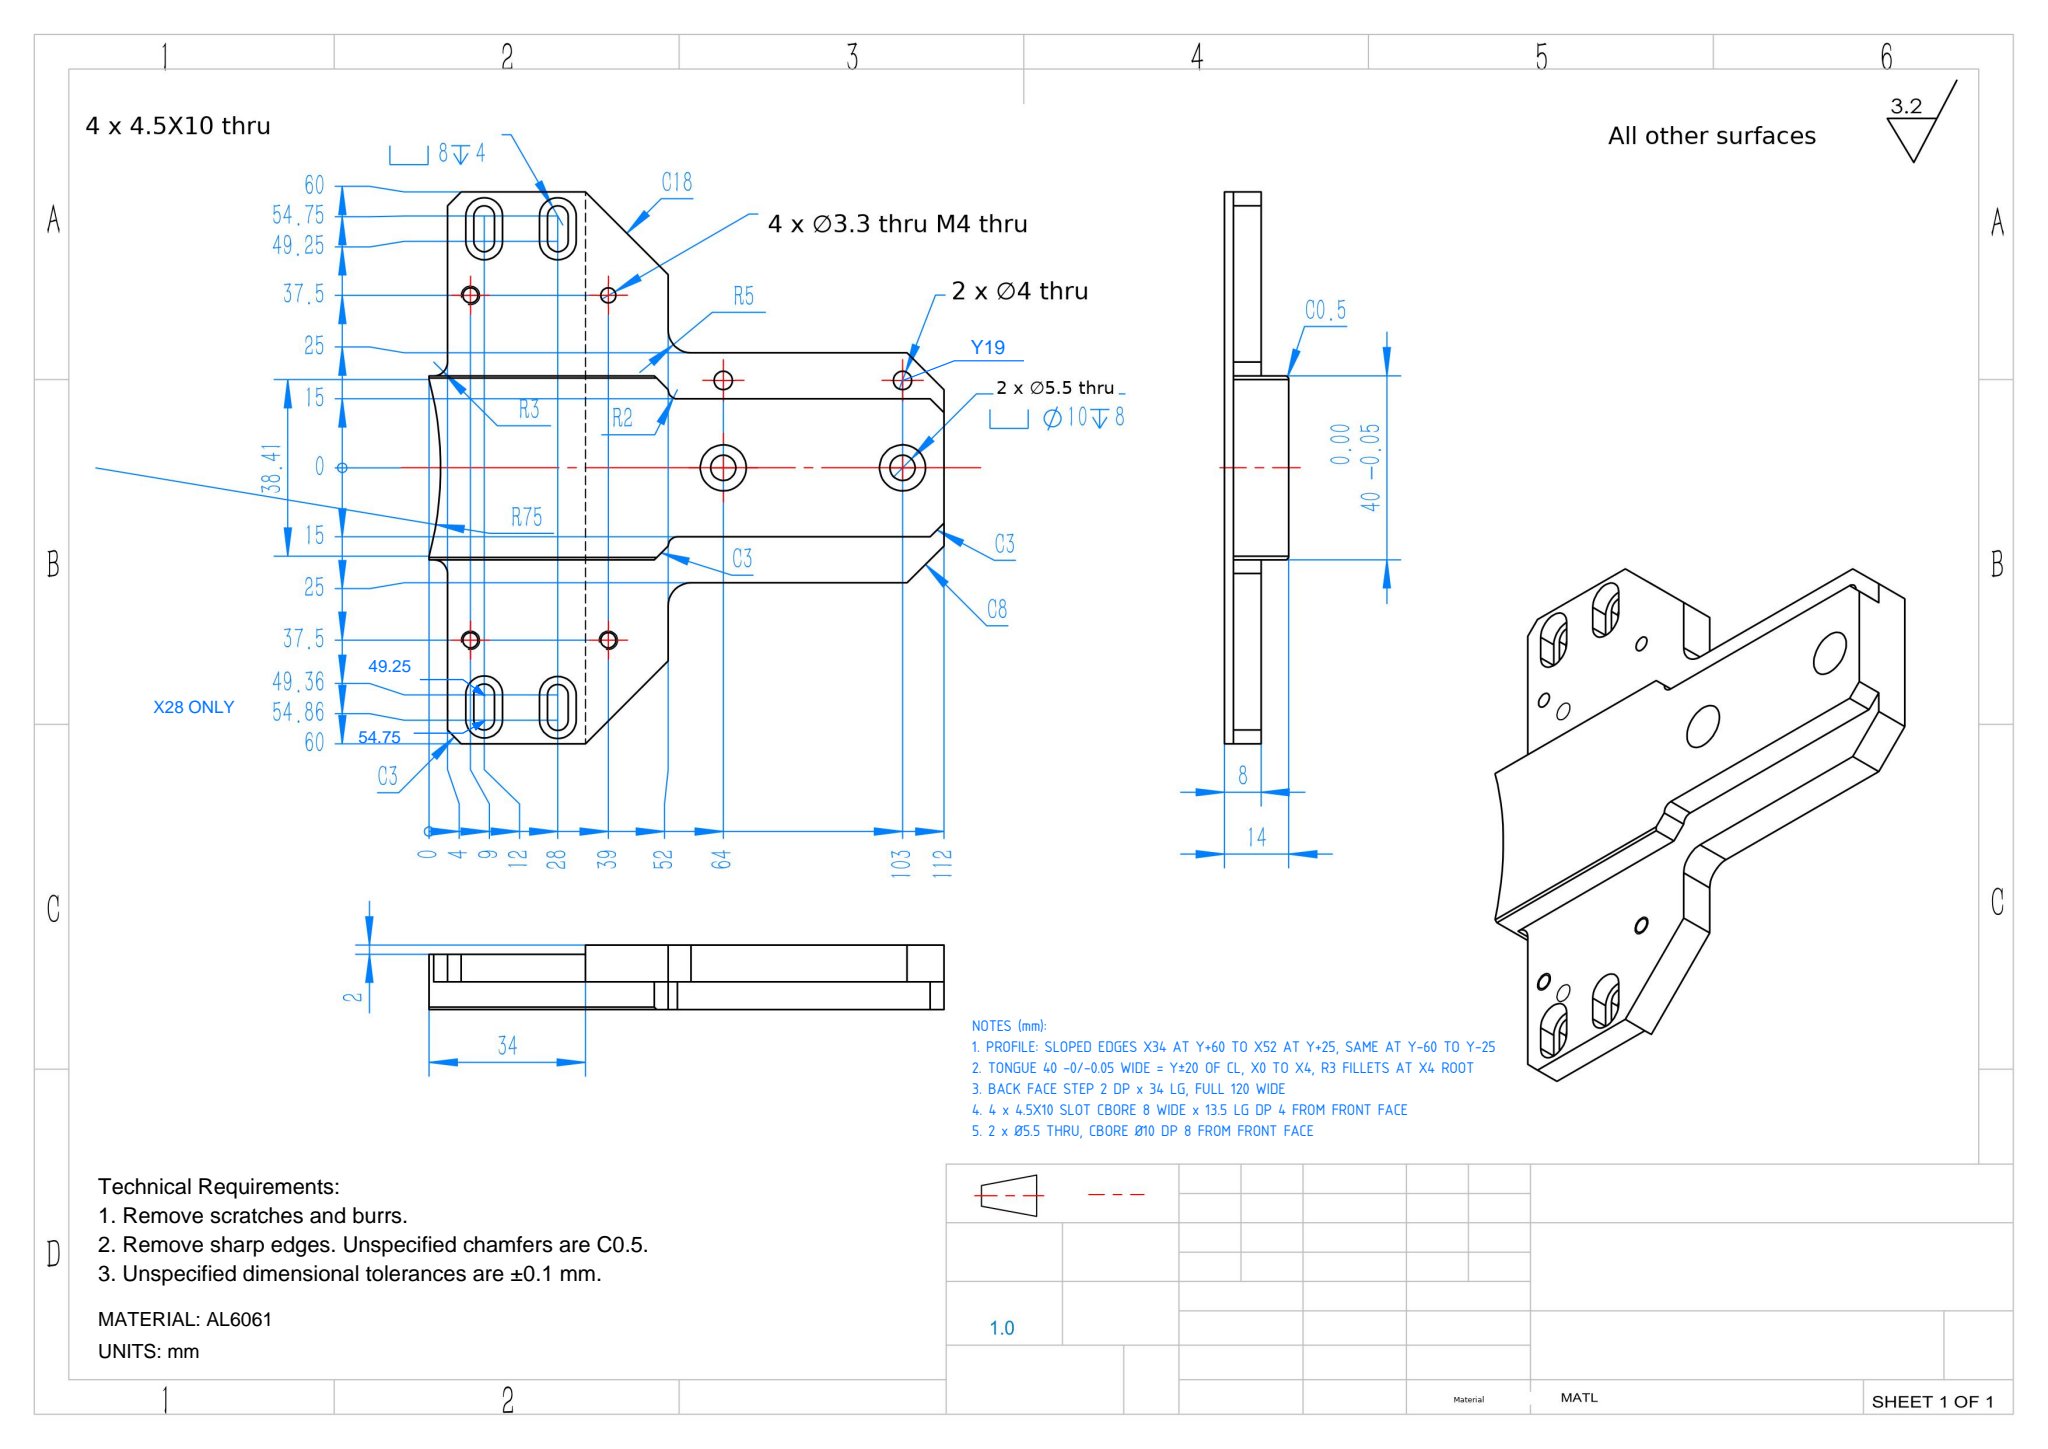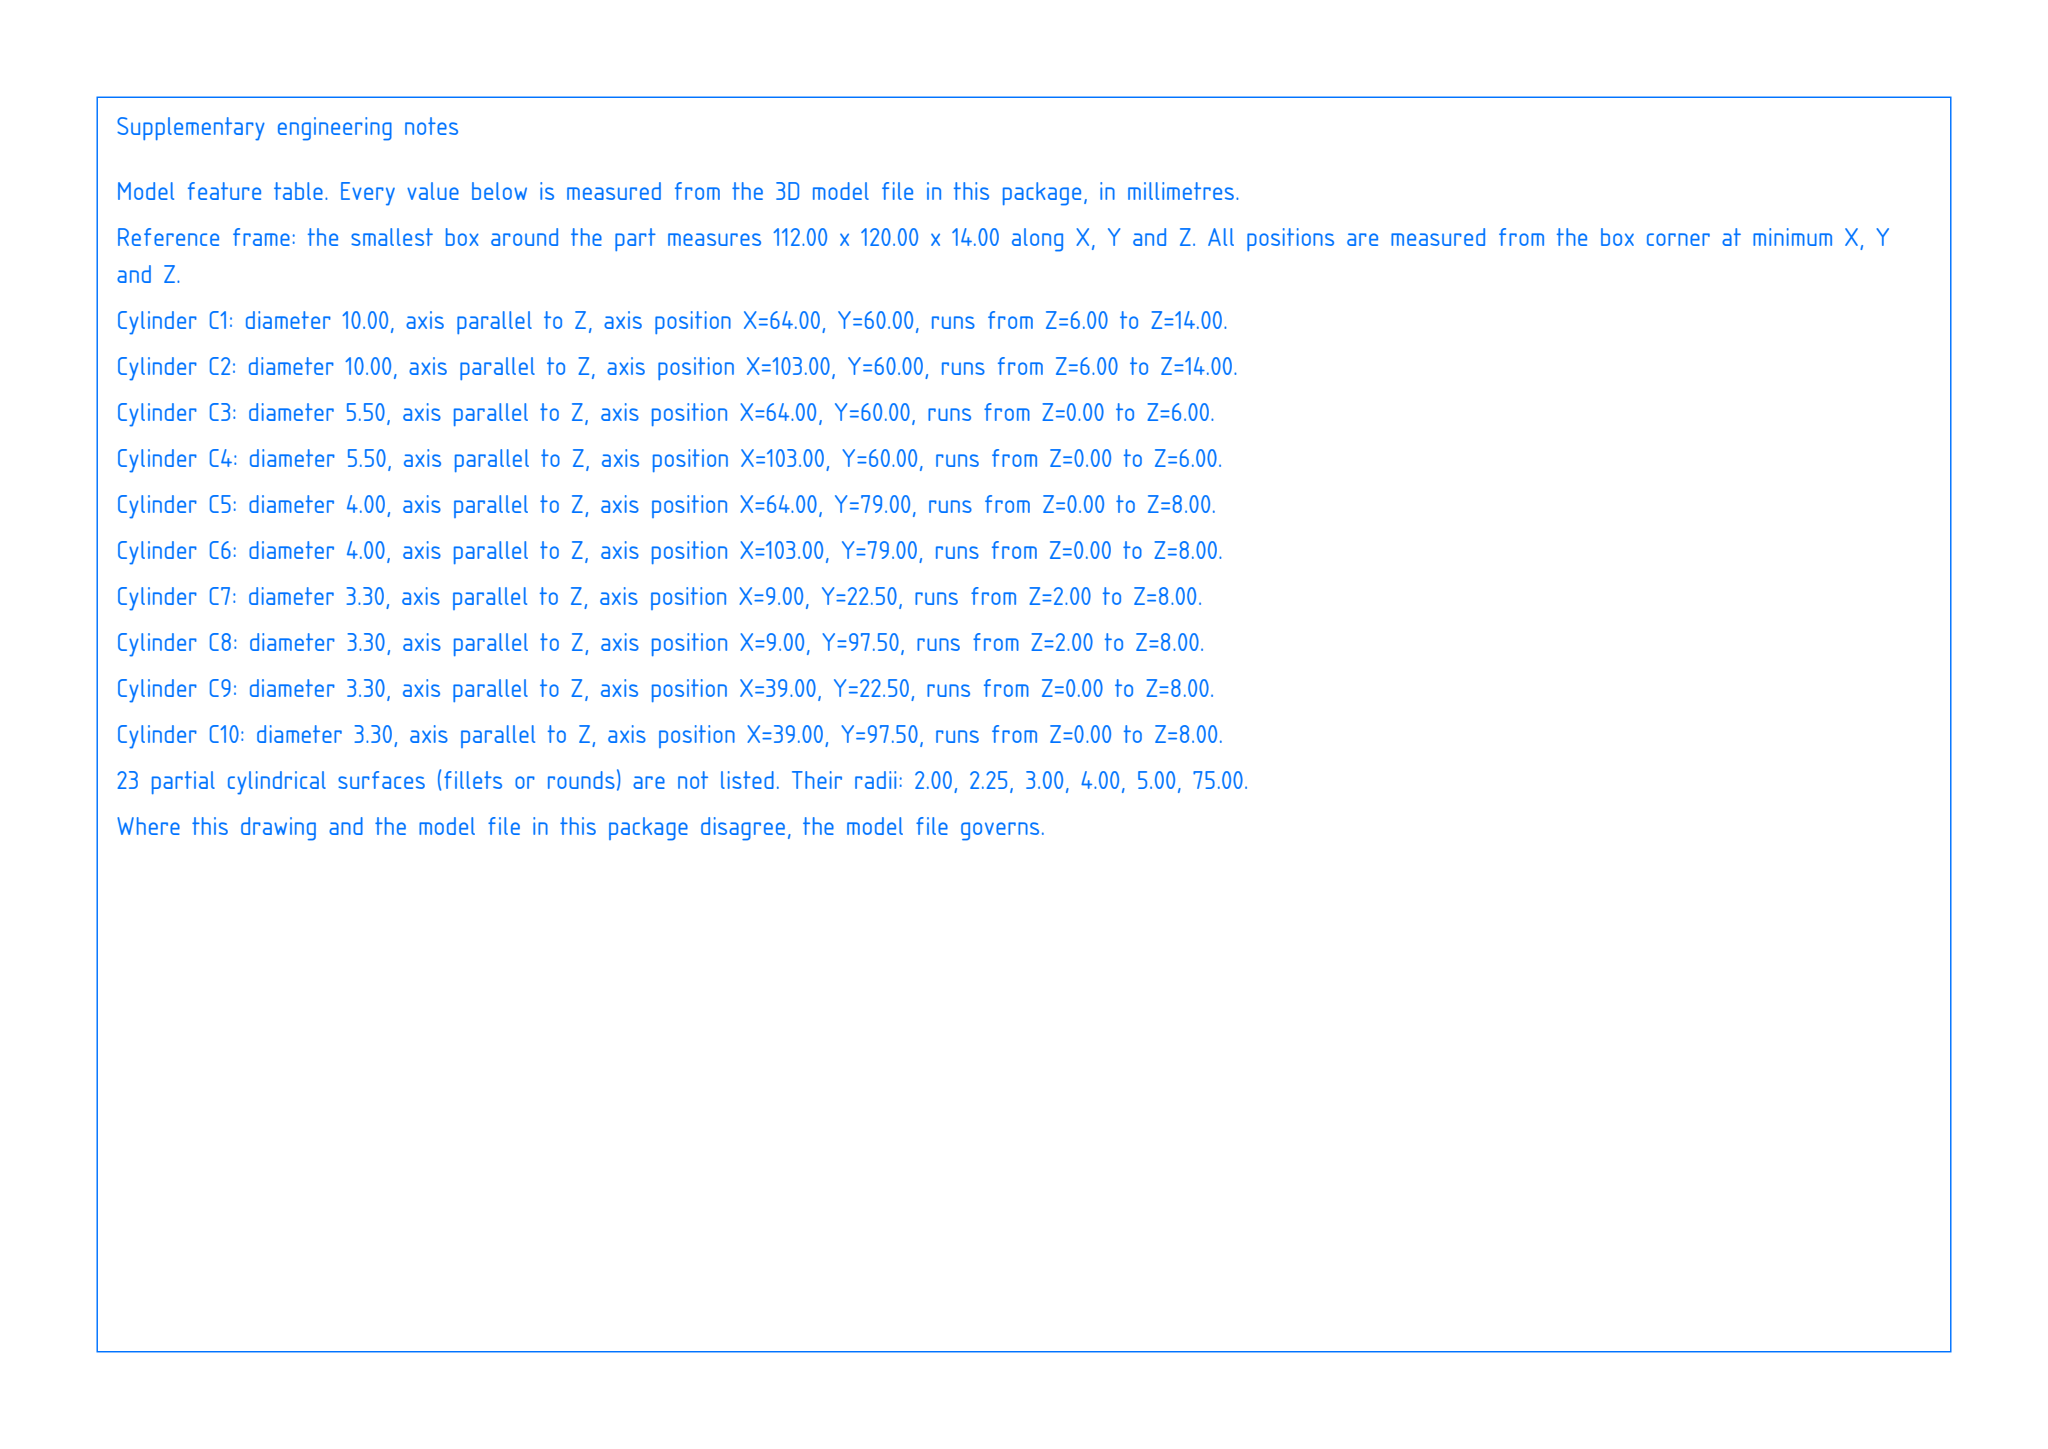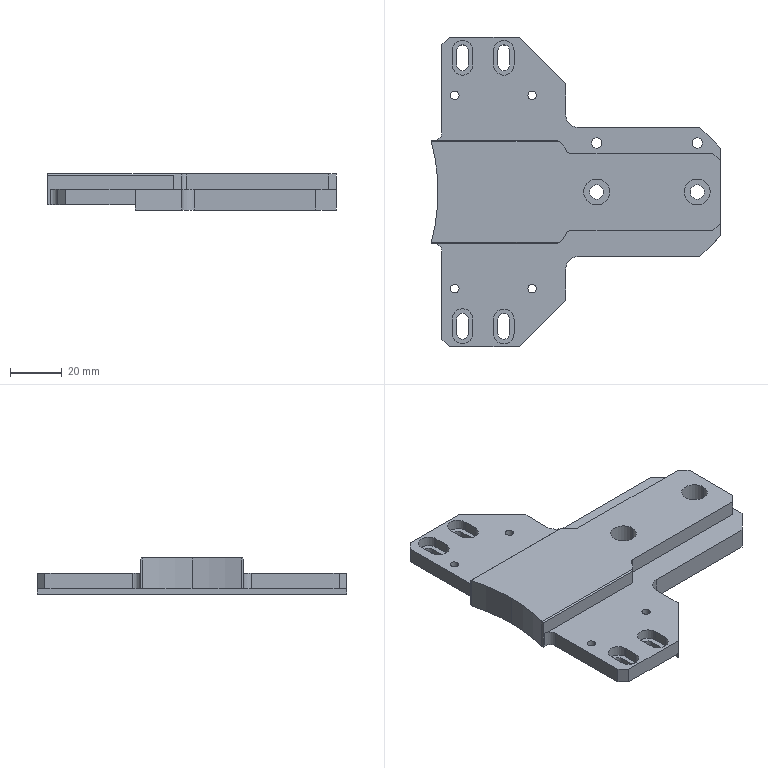Part | SolidWorks | mm | 1 solid | 99 faces | box 112 x 120 x 14 mm | volume 79375 mm3 | plane 55 | cylinder 44 | commonest cylinder face diameters 3.3 x8 4.5 x8 8 x8 4 x6 10 x6 5.5 x4 150 x2 6 x2
Drawing notes:
PROFILE: SLOPED EDGES X34 AT Y+60 TO X52 AT Y+25, SAME AT Y-60 TO Y-25 | from the solid: Planes x=34 / x=52 with y=120 (Y+60), y=85 (Y+25), y=0 (Y-60), y=35 (Y-25) from bbox min; top and bottom edges run 0-34 then slope to the Y±25 faces at x=52
TONGUE 40 -0/-0.05 WIDE = Y±20 OF CL, X0 TO X4, R3 FILLETS AT X4 ROOT | from the solid: y planes 40 and 80 (CL y=60) = ±20; x planes 0 and 4 (2 faces each); R3 fillets = Ø6 cyls at (1,37),(1,83) L=6 tangent to y40/y80 and x4; R75 scallop (Ø150 ctr x-72.5,y60) meets x0 at y40.8/79.2 = 38.41 chord
BACK FACE STEP 2 DP x 34 LG, FULL 120 WIDE | from the solid: z planes 0 and 2 (2 deep), x plane 34 (step end wall), full y 0-120; flange local thk 6 = 4.5 hole L2 + Ø8 c'bore L4
4 x 4.5X10 SLOT CBORE 8 WIDE x 13.5 LG DP 4 FROM FRONT FACE | from the solid: Ø4.5 pairs at (12,5.25/10.75),(12,109.25/114.75),(28,5.14/10.64),(28,109.25/114.75) -> 5.5 c-c, 4.5 wide x 10 lg; Ø8 cyls same centres L=4 -> 8 wide x 13.5 lg; c'bore floor plane z=4 (4 faces), flange z=2..8, so cut from z=8 front face
2 x Ø5.5 THRU, CBORE Ø10 DP 8 FROM FRONT FACE | from the solid: Ø10 L=8 and Ø5.5 L=6 at (64,60) and (103,60); 8+6=14 full thk; c'bore floor plane z=6 (2 faces) -> Ø10 runs z=14 to 6, i.e. from front face